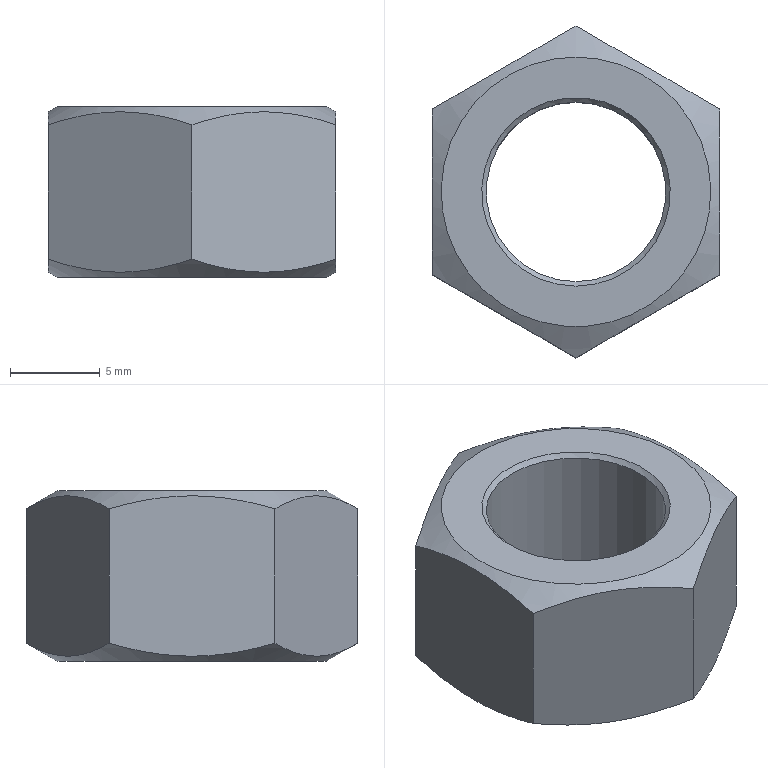Component | NX | GB_T41-2000 | 1 solid | 13 faces | volume 1330 mm3 | plane 8 | cone 4 | cylinder 1 | commonest cylinder face diameters 10 x1